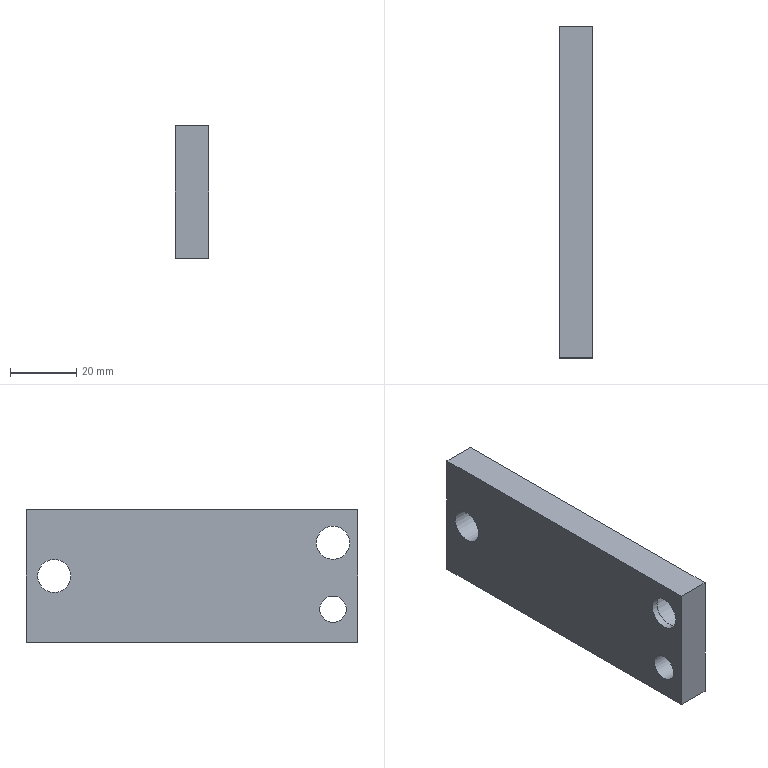Component | NX | DRILL_JIG_PLATE | 1 solid | 13 faces | box 10 x 100 x 40 mm | volume 37387 mm3 | plane 7 | cylinder 5 | cone 1 | commonest cylinder face diameters 10 x2 13 x1 8 x1 4 x1
STEP:
#1=CARTESIAN_POINT('',(0.,0.,0.));
#2=DIRECTION('',(0.,0.,1.));
#3=DIRECTION('',(1.,0.,0.));
#4=AXIS2_PLACEMENT_3D('',#1,#2,#3);
#5=CARTESIAN_POINT('',(49.511,37.872,50.));
#6=VERTEX_POINT('',#5);
#7=CARTESIAN_POINT('',(49.511,37.872,10.));
#8=VERTEX_POINT('',#7);
#9=CARTESIAN_POINT('',(49.511,37.872,50.));
#10=DIRECTION('',(0.,-0.,-1.));
#11=VECTOR('',#10,1.);
#12=LINE('',#9,#11);
#13=CARTESIAN_POINT('',(59.511,37.872,50.));
#14=DIRECTION('',(0.,1.,-0.));
#15=DIRECTION('',(0.,0.,1.));
#16=AXIS2_PLACEMENT_3D('',#13,#14,#15);
#17=PLANE('',#16);
#18=CARTESIAN_POINT('',(0.,-10.));
#19=DIRECTION('',(-1.,0.));
#20=VECTOR('',#19,1.);
#21=LINE('',#18,#20);
#22=(GEOMETRIC_REPRESENTATION_CONTEXT(2)PARAMETRIC_REPRESENTATION_CONTEXT()REPRESENTATION_CONTEXT('',''));
#23=DEFINITIONAL_REPRESENTATION('',(#21),#22);
#24=PCURVE('',#17,#23);
#25=CARTESIAN_POINT('',(49.511,37.872,10.));
#26=DIRECTION('',(1.,0.,0.));
#27=DIRECTION('',(0.,1.,0.));
#28=AXIS2_PLACEMENT_3D('',#25,#26,#27);
#29=PLANE('',#28);
#30=CARTESIAN_POINT('',(0.,40.));
#31=DIRECTION('',(-0.,-1.));
#32=VECTOR('',#31,1.);
#33=LINE('',#30,#32);
#34=(GEOMETRIC_REPRESENTATION_CONTEXT(2)PARAMETRIC_REPRESENTATION_CONTEXT()REPRESENTATION_CONTEXT('',''));
#35=DEFINITIONAL_REPRESENTATION('',(#33),#34);
#36=PCURVE('',#29,#35);
#37=SURFACE_CURVE('',#12,(#24,#36),.PCURVE_S1.);
#38=EDGE_CURVE('',#6,#8,#37,.T.);
#39=ORIENTED_EDGE('',*,*,#38,.T.);
#40=CARTESIAN_POINT('',(59.511,37.872,10.));
#41=VERTEX_POINT('',#40);
#42=CARTESIAN_POINT('',(59.511,37.872,10.));
#43=DIRECTION('',(-1.,0.,0.));
#44=VECTOR('',#43,1.);
#45=LINE('',#42,#44);
#46=CARTESIAN_POINT('',(-40.,0.));
#47=DIRECTION('',(0.,-1.));
#48=VECTOR('',#47,1.);
#49=LINE('',#46,#48);
#50=(GEOMETRIC_REPRESENTATION_CONTEXT(2)PARAMETRIC_REPRESENTATION_CONTEXT()REPRESENTATION_CONTEXT('',''));
#51=DEFINITIONAL_REPRESENTATION('',(#49),#50);
#52=PCURVE('',#17,#51);
#53=CARTESIAN_POINT('',(59.511,37.872,10.));
#54=DIRECTION('',(0.,0.,1.));
#55=DIRECTION('',(1.,0.,0.));
#56=AXIS2_PLACEMENT_3D('',#53,#54,#55);
#57=PLANE('',#56);
#58=CARTESIAN_POINT('',(0.,0.));
#59=DIRECTION('',(-1.,0.));
#60=VECTOR('',#59,1.);
#61=LINE('',#58,#60);
#62=(GEOMETRIC_REPRESENTATION_CONTEXT(2)PARAMETRIC_REPRESENTATION_CONTEXT()REPRESENTATION_CONTEXT('',''));
#63=DEFINITIONAL_REPRESENTATION('',(#61),#62);
#64=PCURVE('',#57,#63);
#65=SURFACE_CURVE('',#45,(#52,#64),.PCURVE_S1.);
#66=EDGE_CURVE('',#41,#8,#65,.T.);
#67=ORIENTED_EDGE('',*,*,#66,.F.);
#68=CARTESIAN_POINT('',(59.511,37.872,50.));
#69=VERTEX_POINT('',#68);
#70=CARTESIAN_POINT('',(59.511,37.872,50.));
#71=DIRECTION('',(0.,-0.,-1.));
#72=VECTOR('',#71,1.);
#73=LINE('',#70,#72);
#74=CARTESIAN_POINT('',(0.,0.));
#75=DIRECTION('',(-1.,0.));
#76=VECTOR('',#75,1.);
#77=LINE('',#74,#76);
#78=(GEOMETRIC_REPRESENTATION_CONTEXT(2)PARAMETRIC_REPRESENTATION_CONTEXT()REPRESENTATION_CONTEXT('',''));
#79=DEFINITIONAL_REPRESENTATION('',(#77),#78);
#80=PCURVE('',#17,#79);
#81=CARTESIAN_POINT('',(59.511,37.872,10.));
#82=DIRECTION('',(1.,0.,0.));
#83=DIRECTION('',(0.,1.,0.));
#84=AXIS2_PLACEMENT_3D('',#81,#82,#83);
#85=PLANE('',#84);
#86=CARTESIAN_POINT('',(0.,40.));
#87=DIRECTION('',(-0.,-1.));
#88=VECTOR('',#87,1.);
#89=LINE('',#86,#88);
#90=(GEOMETRIC_REPRESENTATION_CONTEXT(2)PARAMETRIC_REPRESENTATION_CONTEXT()REPRESENTATION_CONTEXT('',''));
#91=DEFINITIONAL_REPRESENTATION('',(#89),#90);
#92=PCURVE('',#85,#91);
#93=SURFACE_CURVE('',#73,(#80,#92),.PCURVE_S1.);
#94=EDGE_CURVE('',#69,#41,#93,.T.);
#95=ORIENTED_EDGE('',*,*,#94,.F.);
#96=CARTESIAN_POINT('',(59.511,37.872,50.));
#97=DIRECTION('',(-1.,0.,0.));
#98=VECTOR('',#97,1.);
#99=LINE('',#96,#98);
#100=CARTESIAN_POINT('',(0.,0.));
#101=DIRECTION('',(0.,-1.));
#102=VECTOR('',#101,1.);
#103=LINE('',#100,#102);
#104=(GEOMETRIC_REPRESENTATION_CONTEXT(2)PARAMETRIC_REPRESENTATION_CONTEXT()REPRESENTATION_CONTEXT('',''));
#105=DEFINITIONAL_REPRESENTATION('',(#103),#104);
#106=PCURVE('',#17,#105);
#107=CARTESIAN_POINT('',(59.511,137.872,50.));
#108=DIRECTION('',(0.,0.,-1.));
#109=DIRECTION('',(0.,1.,0.));
#110=AXIS2_PLACEMENT_3D('',#107,#108,#109);
#111=PLANE('',#110);
#112=CARTESIAN_POINT('',(-100.,0.));
#113=DIRECTION('',(0.,-1.));
#114=VECTOR('',#113,1.);
#115=LINE('',#112,#114);
#116=(GEOMETRIC_REPRESENTATION_CONTEXT(2)PARAMETRIC_REPRESENTATION_CONTEXT()REPRESENTATION_CONTEXT('',''));
#117=DEFINITIONAL_REPRESENTATION('',(#115),#116);
#118=PCURVE('',#111,#117);
#119=SURFACE_CURVE('',#99,(#106,#118),.PCURVE_S1.);
#120=EDGE_CURVE('',#69,#6,#119,.T.);
#121=ORIENTED_EDGE('',*,*,#120,.T.);
#122=EDGE_LOOP('',(#39,#67,#95,#121));
#123=FACE_BOUND('',#122,.T.);
#124=ADVANCED_FACE('',(#123),#17,.F.);
#125=CARTESIAN_POINT('',(49.511,137.872,10.));
#126=VERTEX_POINT('',#125);
#127=CARTESIAN_POINT('',(49.511,37.872,10.));
#128=DIRECTION('',(0.,1.,0.));
#129=VECTOR('',#128,1.);
#130=LINE('',#127,#129);
#131=CARTESIAN_POINT('',(-10.,0.));
#132=DIRECTION('',(0.,1.));
#133=VECTOR('',#132,1.);
#134=LINE('',#131,#133);
#135=(GEOMETRIC_REPRESENTATION_CONTEXT(2)PARAMETRIC_REPRESENTATION_CONTEXT()REPRESENTATION_CONTEXT('',''));
#136=DEFINITIONAL_REPRESENTATION('',(#134),#135);
#137=PCURVE('',#57,#136);
#138=CARTESIAN_POINT('',(0.,0.));
#139=DIRECTION('',(1.,0.));
#140=VECTOR('',#139,1.);
#141=LINE('',#138,#140);
#142=(GEOMETRIC_REPRESENTATION_CONTEXT(2)PARAMETRIC_REPRESENTATION_CONTEXT()REPRESENTATION_CONTEXT('',''));
#143=DEFINITIONAL_REPRESENTATION('',(#141),#142);
#144=PCURVE('',#29,#143);
#145=SURFACE_CURVE('',#130,(#137,#144),.PCURVE_S1.);
#146=EDGE_CURVE('',#8,#126,#145,.T.);
#147=ORIENTED_EDGE('',*,*,#146,.T.);
#148=CARTESIAN_POINT('',(59.511,137.872,10.));
#149=VERTEX_POINT('',#148);
#150=CARTESIAN_POINT('',(59.511,137.872,10.));
#151=DIRECTION('',(-1.,0.,0.));
#152=VECTOR('',#151,1.);
#153=LINE('',#150,#152);
#154=CARTESIAN_POINT('',(0.,100.));
#155=DIRECTION('',(-1.,0.));
#156=VECTOR('',#155,1.);
#157=LINE('',#154,#156);
#158=(GEOMETRIC_REPRESENTATION_CONTEXT(2)PARAMETRIC_REPRESENTATION_CONTEXT()REPRESENTATION_CONTEXT('',''));
#159=DEFINITIONAL_REPRESENTATION('',(#157),#158);
#160=PCURVE('',#57,#159);
#161=CARTESIAN_POINT('',(59.511,137.872,10.));
#162=DIRECTION('',(0.,-1.,0.));
#163=DIRECTION('',(1.,0.,0.));
#164=AXIS2_PLACEMENT_3D('',#161,#162,#163);
#165=PLANE('',#164);
#166=CARTESIAN_POINT('',(0.,0.));
#167=DIRECTION('',(-1.,0.));
#168=VECTOR('',#167,1.);
#169=LINE('',#166,#168);
#170=(GEOMETRIC_REPRESENTATION_CONTEXT(2)PARAMETRIC_REPRESENTATION_CONTEXT()REPRESENTATION_CONTEXT('',''));
#171=DEFINITIONAL_REPRESENTATION('',(#169),#170);
#172=PCURVE('',#165,#171);
#173=SURFACE_CURVE('',#153,(#160,#172),.PCURVE_S1.);
#174=EDGE_CURVE('',#149,#126,#173,.T.);
#175=ORIENTED_EDGE('',*,*,#174,.F.);
#176=CARTESIAN_POINT('',(59.511,37.872,10.));
#177=DIRECTION('',(0.,1.,0.));
#178=VECTOR('',#177,1.);
#179=LINE('',#176,#178);
#180=CARTESIAN_POINT('',(0.,0.));
#181=DIRECTION('',(0.,1.));
#182=VECTOR('',#181,1.);
#183=LINE('',#180,#182);
#184=(GEOMETRIC_REPRESENTATION_CONTEXT(2)PARAMETRIC_REPRESENTATION_CONTEXT()REPRESENTATION_CONTEXT('',''));
#185=DEFINITIONAL_REPRESENTATION('',(#183),#184);
#186=PCURVE('',#57,#185);
#187=CARTESIAN_POINT('',(0.,0.));
#188=DIRECTION('',(1.,0.));
#189=VECTOR('',#188,1.);
#190=LINE('',#187,#189);
#191=(GEOMETRIC_REPRESENTATION_CONTEXT(2)PARAMETRIC_REPRESENTATION_CONTEXT()REPRESENTATION_CONTEXT('',''));
#192=DEFINITIONAL_REPRESENTATION('',(#190),#191);
#193=PCURVE('',#85,#192);
#194=SURFACE_CURVE('',#179,(#186,#193),.PCURVE_S1.);
#195=EDGE_CURVE('',#41,#149,#194,.T.);
#196=ORIENTED_EDGE('',*,*,#195,.F.);
#197=ORIENTED_EDGE('',*,*,#66,.T.);
#198=EDGE_LOOP('',(#147,#175,#196,#197));
#199=FACE_BOUND('',#198,.T.);
#200=ADVANCED_FACE('',(#199),#57,.F.);
#201=CARTESIAN_POINT('',(49.511,137.872,50.));
#202=VERTEX_POINT('',#201);
#203=CARTESIAN_POINT('',(49.511,137.872,10.));
#204=DIRECTION('',(0.,0.,1.));
#205=VECTOR('',#204,1.);
#206=LINE('',#203,#205);
#207=CARTESIAN_POINT('',(-10.,0.));
#208=DIRECTION('',(0.,1.));
#209=VECTOR('',#208,1.);
#210=LINE('',#207,#209);
#211=(GEOMETRIC_REPRESENTATION_CONTEXT(2)PARAMETRIC_REPRESENTATION_CONTEXT()REPRESENTATION_CONTEXT('',''));
#212=DEFINITIONAL_REPRESENTATION('',(#210),#211);
#213=PCURVE('',#165,#212);
#214=CARTESIAN_POINT('',(100.,0.));
#215=DIRECTION('',(0.,1.));
#216=VECTOR('',#215,1.);
#217=LINE('',#214,#216);
#218=(GEOMETRIC_REPRESENTATION_CONTEXT(2)PARAMETRIC_REPRESENTATION_CONTEXT()REPRESENTATION_CONTEXT('',''));
#219=DEFINITIONAL_REPRESENTATION('',(#217),#218);
#220=PCURVE('',#29,#219);
#221=SURFACE_CURVE('',#206,(#213,#220),.PCURVE_S1.);
#222=EDGE_CURVE('',#126,#202,#221,.T.);
#223=ORIENTED_EDGE('',*,*,#222,.T.);
#224=CARTESIAN_POINT('',(59.511,137.872,50.));
#225=VERTEX_POINT('',#224);
#226=CARTESIAN_POINT('',(59.511,137.872,50.));
#227=DIRECTION('',(-1.,0.,0.));
#228=VECTOR('',#227,1.);
#229=LINE('',#226,#228);
#230=CARTESIAN_POINT('',(0.,40.));
#231=DIRECTION('',(-1.,0.));
#232=VECTOR('',#231,1.);
#233=LINE('',#230,#232);
#234=(GEOMETRIC_REPRESENTATION_CONTEXT(2)PARAMETRIC_REPRESENTATION_CONTEXT()REPRESENTATION_CONTEXT('',''));
#235=DEFINITIONAL_REPRESENTATION('',(#233),#234);
#236=PCURVE('',#165,#235);
#237=CARTESIAN_POINT('',(0.,0.));
#238=DIRECTION('',(0.,-1.));
#239=VECTOR('',#238,1.);
#240=LINE('',#237,#239);
#241=(GEOMETRIC_REPRESENTATION_CONTEXT(2)PARAMETRIC_REPRESENTATION_CONTEXT()REPRESENTATION_CONTEXT('',''));
#242=DEFINITIONAL_REPRESENTATION('',(#240),#241);
#243=PCURVE('',#111,#242);
#244=SURFACE_CURVE('',#229,(#236,#243),.PCURVE_S1.);
#245=EDGE_CURVE('',#225,#202,#244,.T.);
#246=ORIENTED_EDGE('',*,*,#245,.F.);
#247=CARTESIAN_POINT('',(59.511,137.872,10.));
#248=DIRECTION('',(0.,0.,1.));
#249=VECTOR('',#248,1.);
#250=LINE('',#247,#249);
#251=CARTESIAN_POINT('',(0.,0.));
#252=DIRECTION('',(0.,1.));
#253=VECTOR('',#252,1.);
#254=LINE('',#251,#253);
#255=(GEOMETRIC_REPRESENTATION_CONTEXT(2)PARAMETRIC_REPRESENTATION_CONTEXT()REPRESENTATION_CONTEXT('',''));
#256=DEFINITIONAL_REPRESENTATION('',(#254),#255);
#257=PCURVE('',#165,#256);
#258=CARTESIAN_POINT('',(100.,0.));
#259=DIRECTION('',(0.,1.));
#260=VECTOR('',#259,1.);
#261=LINE('',#258,#260);
#262=(GEOMETRIC_REPRESENTATION_CONTEXT(2)PARAMETRIC_REPRESENTATION_CONTEXT()REPRESENTATION_CONTEXT('',''));
#263=DEFINITIONAL_REPRESENTATION('',(#261),#262);
#264=PCURVE('',#85,#263);
#265=SURFACE_CURVE('',#250,(#257,#264),.PCURVE_S1.);
#266=EDGE_CURVE('',#149,#225,#265,.T.);
#267=ORIENTED_EDGE('',*,*,#266,.F.);
#268=ORIENTED_EDGE('',*,*,#174,.T.);
#269=EDGE_LOOP('',(#223,#246,#267,#268));
#270=FACE_BOUND('',#269,.T.);
#271=ADVANCED_FACE('',(#270),#165,.F.);
#272=CARTESIAN_POINT('',(49.511,137.872,50.));
#273=DIRECTION('',(0.,-1.,-0.));
#274=VECTOR('',#273,1.);
#275=LINE('',#272,#274);
#276=CARTESIAN_POINT('',(0.,-10.));
#277=DIRECTION('',(-1.,0.));
#278=VECTOR('',#277,1.);
#279=LINE('',#276,#278);
#280=(GEOMETRIC_REPRESENTATION_CONTEXT(2)PARAMETRIC_REPRESENTATION_CONTEXT()REPRESENTATION_CONTEXT('',''));
#281=DEFINITIONAL_REPRESENTATION('',(#279),#280);
#282=PCURVE('',#111,#281);
#283=CARTESIAN_POINT('',(100.,40.));
#284=DIRECTION('',(-1.,-0.));
#285=VECTOR('',#284,1.);
#286=LINE('',#283,#285);
#287=(GEOMETRIC_REPRESENTATION_CONTEXT(2)PARAMETRIC_REPRESENTATION_CONTEXT()REPRESENTATION_CONTEXT('',''));
#288=DEFINITIONAL_REPRESENTATION('',(#286),#287);
#289=PCURVE('',#29,#288);
#290=SURFACE_CURVE('',#275,(#282,#289),.PCURVE_S1.);
#291=EDGE_CURVE('',#202,#6,#290,.T.);
#292=ORIENTED_EDGE('',*,*,#291,.T.);
#293=ORIENTED_EDGE('',*,*,#120,.F.);
#294=CARTESIAN_POINT('',(59.511,137.872,50.));
#295=DIRECTION('',(0.,-1.,-0.));
#296=VECTOR('',#295,1.);
#297=LINE('',#294,#296);
#298=CARTESIAN_POINT('',(0.,0.));
#299=DIRECTION('',(-1.,0.));
#300=VECTOR('',#299,1.);
#301=LINE('',#298,#300);
#302=(GEOMETRIC_REPRESENTATION_CONTEXT(2)PARAMETRIC_REPRESENTATION_CONTEXT()REPRESENTATION_CONTEXT('',''));
#303=DEFINITIONAL_REPRESENTATION('',(#301),#302);
#304=PCURVE('',#111,#303);
#305=CARTESIAN_POINT('',(100.,40.));
#306=DIRECTION('',(-1.,-0.));
#307=VECTOR('',#306,1.);
#308=LINE('',#305,#307);
#309=(GEOMETRIC_REPRESENTATION_CONTEXT(2)PARAMETRIC_REPRESENTATION_CONTEXT()REPRESENTATION_CONTEXT('',''));
#310=DEFINITIONAL_REPRESENTATION('',(#308),#309);
#311=PCURVE('',#85,#310);
#312=SURFACE_CURVE('',#297,(#304,#311),.PCURVE_S1.);
#313=EDGE_CURVE('',#225,#69,#312,.T.);
#314=ORIENTED_EDGE('',*,*,#313,.F.);
#315=ORIENTED_EDGE('',*,*,#245,.T.);
#316=EDGE_LOOP('',(#292,#293,#314,#315));
#317=FACE_BOUND('',#316,.T.);
#318=ADVANCED_FACE('',(#317),#111,.F.);
#319=CARTESIAN_POINT('',(59.511,117.396,30.));
#320=VERTEX_POINT('',#319);
#321=CARTESIAN_POINT('',(59.511,119.396,30.));
#322=DIRECTION('',(-1.,0.,0.));
#323=DIRECTION('',(0.,-1.,0.));
#324=AXIS2_PLACEMENT_3D('',#321,#322,#323);
#325=CIRCLE('',#324,2.);
#326=CARTESIAN_POINT('',(79.524,20.));
#327=CARTESIAN_POINT('',(79.524,23.464));
#328=CARTESIAN_POINT('',(82.524,21.732));
#329=CARTESIAN_POINT('',(85.524,20.));
#330=CARTESIAN_POINT('',(82.524,18.268));
#331=CARTESIAN_POINT('',(79.524,16.536));
#332=CARTESIAN_POINT('',(79.524,20.));
#333=(BOUNDED_CURVE()B_SPLINE_CURVE(2,(#326,#327,#328,#329,#330,#331,#332),.UNSPECIFIED.,.T.,.F.)B_SPLINE_CURVE_WITH_KNOTS((1,2,2,2,2,1),(-2.094,0.,2.094,4.189,6.283,8.378),.UNSPECIFIED.)CURVE()GEOMETRIC_REPRESENTATION_ITEM()RATIONAL_B_SPLINE_CURVE((1.,0.5,1.,0.5,1.,0.5,1.))REPRESENTATION_ITEM(''));
#334=(GEOMETRIC_REPRESENTATION_CONTEXT(2)PARAMETRIC_REPRESENTATION_CONTEXT()REPRESENTATION_CONTEXT('',''));
#335=DEFINITIONAL_REPRESENTATION('',(#333),#334);
#336=PCURVE('',#85,#335);
#337=CARTESIAN_POINT('',(59.511,119.396,30.));
#338=DIRECTION('',(-1.,0.,0.));
#339=DIRECTION('',(0.,-1.,0.));
#340=AXIS2_PLACEMENT_3D('',#337,#338,#339);
#341=CYLINDRICAL_SURFACE('',#340,2.);
#342=CARTESIAN_POINT('',(0.,0.));
#343=DIRECTION('',(1.,0.));
#344=VECTOR('',#343,1.);
#345=LINE('',#342,#344);
#346=(GEOMETRIC_REPRESENTATION_CONTEXT(2)PARAMETRIC_REPRESENTATION_CONTEXT()REPRESENTATION_CONTEXT('',''));
#347=DEFINITIONAL_REPRESENTATION('',(#345),#346);
#348=PCURVE('',#341,#347);
#349=SURFACE_CURVE('',#325,(#336,#348),.PCURVE_S1.);
#350=EDGE_CURVE('',#320,#320,#349,.T.);
#351=ORIENTED_EDGE('',*,*,#350,.T.);
#352=EDGE_LOOP('',(#351));
#353=FACE_BOUND('',#352,.T.);
#354=CARTESIAN_POINT('',(59.511,134.396,30.));
#355=VERTEX_POINT('',#354);
#356=CARTESIAN_POINT('',(59.511,129.396,30.));
#357=DIRECTION('',(1.,0.,0.));
#358=DIRECTION('',(0.,1.,0.));
#359=AXIS2_PLACEMENT_3D('',#356,#357,#358);
#360=CIRCLE('',#359,5.);
#361=CARTESIAN_POINT('',(91.524,20.));
#362=DIRECTION('',(1.,0.));
#363=AXIS2_PLACEMENT_2D('',#361,#362);
#364=CIRCLE('',#363,5.);
#365=(GEOMETRIC_REPRESENTATION_CONTEXT(2)PARAMETRIC_REPRESENTATION_CONTEXT()REPRESENTATION_CONTEXT('',''));
#366=DEFINITIONAL_REPRESENTATION('',(#364),#365);
#367=PCURVE('',#85,#366);
#368=CARTESIAN_POINT('',(14.511,129.396,30.));
#369=DIRECTION('',(1.,0.,0.));
#370=DIRECTION('',(0.,1.,0.));
#371=AXIS2_PLACEMENT_3D('',#368,#369,#370);
#372=CYLINDRICAL_SURFACE('',#371,5.);
#373=CARTESIAN_POINT('',(0.,45.));
#374=DIRECTION('',(1.,0.));
#375=VECTOR('',#374,1.);
#376=LINE('',#373,#375);
#377=(GEOMETRIC_REPRESENTATION_CONTEXT(2)PARAMETRIC_REPRESENTATION_CONTEXT()REPRESENTATION_CONTEXT('',''));
#378=DEFINITIONAL_REPRESENTATION('',(#376),#377);
#379=PCURVE('',#372,#378);
#380=SURFACE_CURVE('',#360,(#367,#379),.PCURVE_S1.);
#381=EDGE_CURVE('',#355,#355,#380,.T.);
#382=ORIENTED_EDGE('',*,*,#381,.F.);
#383=EDGE_LOOP('',(#382));
#384=FACE_BOUND('',#383,.T.);
#385=CARTESIAN_POINT('',(59.511,49.372,20.));
#386=VERTEX_POINT('',#385);
#387=CARTESIAN_POINT('',(59.511,45.372,20.));
#388=DIRECTION('',(1.,0.,0.));
#389=DIRECTION('',(0.,1.,0.));
#390=AXIS2_PLACEMENT_3D('',#387,#388,#389);
#391=CIRCLE('',#390,4.);
#392=CARTESIAN_POINT('',(7.5,10.));
#393=DIRECTION('',(1.,0.));
#394=AXIS2_PLACEMENT_2D('',#392,#393);
#395=CIRCLE('',#394,4.);
#396=(GEOMETRIC_REPRESENTATION_CONTEXT(2)PARAMETRIC_REPRESENTATION_CONTEXT()REPRESENTATION_CONTEXT('',''));
#397=DEFINITIONAL_REPRESENTATION('',(#395),#396);
#398=PCURVE('',#85,#397);
#399=CARTESIAN_POINT('',(14.511,45.372,20.));
#400=DIRECTION('',(1.,0.,0.));
#401=DIRECTION('',(0.,1.,0.));
#402=AXIS2_PLACEMENT_3D('',#399,#400,#401);
#403=CYLINDRICAL_SURFACE('',#402,4.);
#404=CARTESIAN_POINT('',(0.,45.));
#405=DIRECTION('',(1.,0.));
#406=VECTOR('',#405,1.);
#407=LINE('',#404,#406);
#408=(GEOMETRIC_REPRESENTATION_CONTEXT(2)PARAMETRIC_REPRESENTATION_CONTEXT()REPRESENTATION_CONTEXT('',''));
#409=DEFINITIONAL_REPRESENTATION('',(#407),#408);
#410=PCURVE('',#403,#409);
#411=SURFACE_CURVE('',#391,(#398,#410),.PCURVE_S1.);
#412=EDGE_CURVE('',#386,#386,#411,.T.);
#413=ORIENTED_EDGE('',*,*,#412,.F.);
#414=EDGE_LOOP('',(#413));
#415=FACE_BOUND('',#414,.T.);
#416=CARTESIAN_POINT('',(59.511,38.872,40.));
#417=VERTEX_POINT('',#416);
#418=CARTESIAN_POINT('',(59.511,45.372,40.));
#419=DIRECTION('',(-1.,0.,0.));
#420=DIRECTION('',(0.,-1.,0.));
#421=AXIS2_PLACEMENT_3D('',#418,#419,#420);
#422=CIRCLE('',#421,6.5);
#423=CARTESIAN_POINT('',(1.,30.));
#424=CARTESIAN_POINT('',(1.,41.258));
#425=CARTESIAN_POINT('',(10.75,35.629));
#426=CARTESIAN_POINT('',(20.5,30.));
#427=CARTESIAN_POINT('',(10.75,24.371));
#428=CARTESIAN_POINT('',(1.,18.742));
#429=CARTESIAN_POINT('',(1.,30.));
#430=(BOUNDED_CURVE()B_SPLINE_CURVE(2,(#423,#424,#425,#426,#427,#428,#429),.UNSPECIFIED.,.T.,.F.)B_SPLINE_CURVE_WITH_KNOTS((1,2,2,2,2,1),(-2.094,0.,2.094,4.189,6.283,8.378),.UNSPECIFIED.)CURVE()GEOMETRIC_REPRESENTATION_ITEM()RATIONAL_B_SPLINE_CURVE((1.,0.5,1.,0.5,1.,0.5,1.))REPRESENTATION_ITEM(''));
#431=(GEOMETRIC_REPRESENTATION_CONTEXT(2)PARAMETRIC_REPRESENTATION_CONTEXT()REPRESENTATION_CONTEXT('',''));
#432=DEFINITIONAL_REPRESENTATION('',(#430),#431);
#433=PCURVE('',#85,#432);
#434=CARTESIAN_POINT('',(59.511,45.372,40.));
#435=DIRECTION('',(-1.,0.,0.));
#436=DIRECTION('',(0.,-1.,0.));
#437=AXIS2_PLACEMENT_3D('',#434,#435,#436);
#438=CYLINDRICAL_SURFACE('',#437,6.5);
#439=CARTESIAN_POINT('',(0.,0.));
#440=DIRECTION('',(1.,0.));
#441=VECTOR('',#440,1.);
#442=LINE('',#439,#441);
#443=(GEOMETRIC_REPRESENTATION_CONTEXT(2)PARAMETRIC_REPRESENTATION_CONTEXT()REPRESENTATION_CONTEXT('',''));
#444=DEFINITIONAL_REPRESENTATION('',(#442),#443);
#445=PCURVE('',#438,#444);
#446=SURFACE_CURVE('',#422,(#433,#445),.PCURVE_S1.);
#447=EDGE_CURVE('',#417,#417,#446,.T.);
#448=ORIENTED_EDGE('',*,*,#447,.T.);
#449=EDGE_LOOP('',(#448));
#450=FACE_BOUND('',#449,.T.);
#451=ORIENTED_EDGE('',*,*,#94,.T.);
#452=ORIENTED_EDGE('',*,*,#195,.T.);
#453=ORIENTED_EDGE('',*,*,#266,.T.);
#454=ORIENTED_EDGE('',*,*,#313,.T.);
#455=EDGE_LOOP('',(#451,#452,#453,#454));
#456=FACE_BOUND('',#455,.T.);
#457=ADVANCED_FACE('',(#353,#384,#415,#450,#456),#85,.T.);
#458=CARTESIAN_POINT('',(49.511,134.396,30.));
#459=VERTEX_POINT('',#458);
#460=CARTESIAN_POINT('',(49.511,129.396,30.));
#461=DIRECTION('',(1.,0.,0.));
#462=DIRECTION('',(0.,1.,0.));
#463=AXIS2_PLACEMENT_3D('',#460,#461,#462);
#464=CIRCLE('',#463,5.);
#465=CARTESIAN_POINT('',(91.524,20.));
#466=DIRECTION('',(1.,0.));
#467=AXIS2_PLACEMENT_2D('',#465,#466);
#468=CIRCLE('',#467,5.);
#469=(GEOMETRIC_REPRESENTATION_CONTEXT(2)PARAMETRIC_REPRESENTATION_CONTEXT()REPRESENTATION_CONTEXT('',''));
#470=DEFINITIONAL_REPRESENTATION('',(#468),#469);
#471=PCURVE('',#29,#470);
#472=CARTESIAN_POINT('',(0.,35.));
#473=DIRECTION('',(1.,0.));
#474=VECTOR('',#473,1.);
#475=LINE('',#472,#474);
#476=(GEOMETRIC_REPRESENTATION_CONTEXT(2)PARAMETRIC_REPRESENTATION_CONTEXT()REPRESENTATION_CONTEXT('',''));
#477=DEFINITIONAL_REPRESENTATION('',(#475),#476);
#478=PCURVE('',#372,#477);
#479=SURFACE_CURVE('',#464,(#471,#478),.PCURVE_S1.);
#480=EDGE_CURVE('',#459,#459,#479,.T.);
#481=ORIENTED_EDGE('',*,*,#480,.T.);
#482=EDGE_LOOP('',(#481));
#483=FACE_BOUND('',#482,.T.);
#484=CARTESIAN_POINT('',(49.511,49.372,20.));
#485=VERTEX_POINT('',#484);
#486=CARTESIAN_POINT('',(49.511,45.372,20.));
#487=DIRECTION('',(1.,0.,0.));
#488=DIRECTION('',(0.,1.,0.));
#489=AXIS2_PLACEMENT_3D('',#486,#487,#488);
#490=CIRCLE('',#489,4.);
#491=CARTESIAN_POINT('',(7.5,10.));
#492=DIRECTION('',(1.,0.));
#493=AXIS2_PLACEMENT_2D('',#491,#492);
#494=CIRCLE('',#493,4.);
#495=(GEOMETRIC_REPRESENTATION_CONTEXT(2)PARAMETRIC_REPRESENTATION_CONTEXT()REPRESENTATION_CONTEXT('',''));
#496=DEFINITIONAL_REPRESENTATION('',(#494),#495);
#497=PCURVE('',#29,#496);
#498=CARTESIAN_POINT('',(0.,35.));
#499=DIRECTION('',(1.,0.));
#500=VECTOR('',#499,1.);
#501=LINE('',#498,#500);
#502=(GEOMETRIC_REPRESENTATION_CONTEXT(2)PARAMETRIC_REPRESENTATION_CONTEXT()REPRESENTATION_CONTEXT('',''));
#503=DEFINITIONAL_REPRESENTATION('',(#501),#502);
#504=PCURVE('',#403,#503);
#505=SURFACE_CURVE('',#490,(#497,#504),.PCURVE_S1.);
#506=EDGE_CURVE('',#485,#485,#505,.T.);
#507=ORIENTED_EDGE('',*,*,#506,.T.);
#508=EDGE_LOOP('',(#507));
#509=FACE_BOUND('',#508,.T.);
#510=CARTESIAN_POINT('',(49.511,50.372,40.));
#511=VERTEX_POINT('',#510);
#512=CARTESIAN_POINT('',(49.511,40.372,40.));
#513=VERTEX_POINT('',#512);
#514=CARTESIAN_POINT('',(49.511,45.372,40.));
#515=DIRECTION('',(1.,0.,0.));
#516=DIRECTION('',(0.,1.,0.));
#517=AXIS2_PLACEMENT_3D('',#514,#515,#516);
#518=CIRCLE('',#517,5.);
#519=CARTESIAN_POINT('',(7.5,30.));
#520=DIRECTION('',(1.,0.));
#521=AXIS2_PLACEMENT_2D('',#519,#520);
#522=CIRCLE('',#521,5.);
#523=(GEOMETRIC_REPRESENTATION_CONTEXT(2)PARAMETRIC_REPRESENTATION_CONTEXT()REPRESENTATION_CONTEXT('',''));
#524=DEFINITIONAL_REPRESENTATION('',(#522),#523);
#525=PCURVE('',#29,#524);
#526=CARTESIAN_POINT('',(39.511,45.372,40.));
#527=DIRECTION('',(-1.,0.,0.));
#528=DIRECTION('',(0.,-1.,0.));
#529=AXIS2_PLACEMENT_3D('',#526,#527,#528);
#530=CYLINDRICAL_SURFACE('',#529,5.);
#531=CARTESIAN_POINT('',(3.142,-10.));
#532=DIRECTION('',(-1.,0.));
#533=VECTOR('',#532,1.);
#534=LINE('',#531,#533);
#535=(GEOMETRIC_REPRESENTATION_CONTEXT(2)PARAMETRIC_REPRESENTATION_CONTEXT()REPRESENTATION_CONTEXT('',''));
#536=DEFINITIONAL_REPRESENTATION('',(#534),#535);
#537=PCURVE('',#530,#536);
#538=SURFACE_CURVE('',#518,(#525,#537),.PCURVE_S1.);
#539=EDGE_CURVE('',#511,#513,#538,.T.);
#540=ORIENTED_EDGE('',*,*,#539,.T.);
#541=CARTESIAN_POINT('',(49.511,45.372,40.));
#542=DIRECTION('',(1.,0.,0.));
#543=DIRECTION('',(0.,1.,0.));
#544=AXIS2_PLACEMENT_3D('',#541,#542,#543);
#545=CIRCLE('',#544,5.);
#546=CARTESIAN_POINT('',(7.5,30.));
#547=DIRECTION('',(1.,0.));
#548=AXIS2_PLACEMENT_2D('',#546,#547);
#549=CIRCLE('',#548,5.);
#550=(GEOMETRIC_REPRESENTATION_CONTEXT(2)PARAMETRIC_REPRESENTATION_CONTEXT()REPRESENTATION_CONTEXT('',''));
#551=DEFINITIONAL_REPRESENTATION('',(#549),#550);
#552=PCURVE('',#29,#551);
#553=CARTESIAN_POINT('',(9.425,-10.));
#554=DIRECTION('',(-1.,0.));
#555=VECTOR('',#554,1.);
#556=LINE('',#553,#555);
#557=(GEOMETRIC_REPRESENTATION_CONTEXT(2)PARAMETRIC_REPRESENTATION_CONTEXT()REPRESENTATION_CONTEXT('',''));
#558=DEFINITIONAL_REPRESENTATION('',(#556),#557);
#559=PCURVE('',#530,#558);
#560=SURFACE_CURVE('',#545,(#552,#559),.PCURVE_S1.);
#561=EDGE_CURVE('',#513,#511,#560,.T.);
#562=ORIENTED_EDGE('',*,*,#561,.T.);
#563=EDGE_LOOP('',(#540,#562));
#564=FACE_BOUND('',#563,.T.);
#565=ORIENTED_EDGE('',*,*,#38,.F.);
#566=ORIENTED_EDGE('',*,*,#291,.F.);
#567=ORIENTED_EDGE('',*,*,#222,.F.);
#568=ORIENTED_EDGE('',*,*,#146,.F.);
#569=EDGE_LOOP('',(#565,#566,#567,#568));
#570=FACE_BOUND('',#569,.T.);
#571=ADVANCED_FACE('',(#483,#509,#564,#570),#29,.F.);
#572=CARTESIAN_POINT('',(51.511,40.372,40.));
#573=VERTEX_POINT('',#572);
#574=CARTESIAN_POINT('',(51.511,45.372,40.));
#575=DIRECTION('',(1.,0.,0.));
#576=DIRECTION('',(0.,-1.,0.));
#577=AXIS2_PLACEMENT_3D('',#574,#575,#576);
#578=CIRCLE('',#577,5.);
#579=CARTESIAN_POINT('',(6.283,-12.));
#580=DIRECTION('',(-1.,0.));
#581=VECTOR('',#580,1.);
#582=LINE('',#579,#581);
#583=(GEOMETRIC_REPRESENTATION_CONTEXT(2)PARAMETRIC_REPRESENTATION_CONTEXT()REPRESENTATION_CONTEXT('',''));
#584=DEFINITIONAL_REPRESENTATION('',(#582),#583);
#585=PCURVE('',#530,#584);
#586=CARTESIAN_POINT('',(51.511,45.372,40.));
#587=DIRECTION('',(-1.,0.,0.));
#588=DIRECTION('',(0.,-1.,0.));
#589=AXIS2_PLACEMENT_3D('',#586,#587,#588);
#590=PLANE('',#589);
#591=CARTESIAN_POINT('',(5.,0.));
#592=CARTESIAN_POINT('',(5.,-8.66));
#593=CARTESIAN_POINT('',(-2.5,-4.33));
#594=CARTESIAN_POINT('',(-10.,-0.));
#595=CARTESIAN_POINT('',(-2.5,4.33));
#596=CARTESIAN_POINT('',(5.,8.66));
#597=CARTESIAN_POINT('',(5.,0.));
#598=(BOUNDED_CURVE()B_SPLINE_CURVE(2,(#591,#592,#593,#594,#595,#596,#597),.UNSPECIFIED.,.T.,.F.)B_SPLINE_CURVE_WITH_KNOTS((1,2,2,2,2,1),(-2.094,0.,2.094,4.189,6.283,8.378),.UNSPECIFIED.)CURVE()GEOMETRIC_REPRESENTATION_ITEM()RATIONAL_B_SPLINE_CURVE((1.,0.5,1.,0.5,1.,0.5,1.))REPRESENTATION_ITEM(''));
#599=(GEOMETRIC_REPRESENTATION_CONTEXT(2)PARAMETRIC_REPRESENTATION_CONTEXT()REPRESENTATION_CONTEXT('',''));
#600=DEFINITIONAL_REPRESENTATION('',(#598),#599);
#601=PCURVE('',#590,#600);
#602=SURFACE_CURVE('',#578,(#585,#601),.PCURVE_S1.);
#603=EDGE_CURVE('',#573,#573,#602,.T.);
#604=ORIENTED_EDGE('',*,*,#603,.F.);
#605=CARTESIAN_POINT('',(51.511,40.372,40.));
#606=CARTESIAN_POINT('',(49.511,40.372,40.));
#607=B_SPLINE_CURVE_WITH_KNOTS('',1,(#605,#606),.UNSPECIFIED.,.F.,.F.,(2,2),(-12.,-10.),.PIECEWISE_BEZIER_KNOTS.);
#608=CARTESIAN_POINT('',(6.283,0.));
#609=DIRECTION('',(0.,1.));
#610=VECTOR('',#609,1.);
#611=LINE('',#608,#610);
#612=(GEOMETRIC_REPRESENTATION_CONTEXT(2)PARAMETRIC_REPRESENTATION_CONTEXT()REPRESENTATION_CONTEXT('',''));
#613=DEFINITIONAL_REPRESENTATION('',(#611),#612);
#614=PCURVE('',#530,#613);
#615=CARTESIAN_POINT('',(0.,0.));
#616=DIRECTION('',(0.,1.));
#617=VECTOR('',#616,1.);
#618=LINE('',#615,#617);
#619=(GEOMETRIC_REPRESENTATION_CONTEXT(2)PARAMETRIC_REPRESENTATION_CONTEXT()REPRESENTATION_CONTEXT('',''));
#620=DEFINITIONAL_REPRESENTATION('',(#618),#619);
#621=PCURVE('',#530,#620);
#622=SEAM_CURVE('',#607,(#614,#621),.PCURVE_S1.);
#623=EDGE_CURVE('',#573,#513,#622,.T.);
#624=ORIENTED_EDGE('',*,*,#623,.T.);
#625=ORIENTED_EDGE('',*,*,#561,.T.);
#626=ORIENTED_EDGE('',*,*,#539,.T.);
#627=ORIENTED_EDGE('',*,*,#623,.F.);
#628=EDGE_LOOP('',(#604,#624,#625,#626,#627));
#629=FACE_BOUND('',#628,.F.);
#630=ADVANCED_FACE('',(#629),#530,.F.);
#631=ORIENTED_EDGE('',*,*,#603,.F.);
#632=EDGE_LOOP('',(#631));
#633=FACE_BOUND('',#632,.T.);
#634=CARTESIAN_POINT('',(51.511,38.872,40.));
#635=VERTEX_POINT('',#634);
#636=CARTESIAN_POINT('',(51.511,45.372,40.));
#637=DIRECTION('',(1.,0.,0.));
#638=DIRECTION('',(0.,-1.,0.));
#639=AXIS2_PLACEMENT_3D('',#636,#637,#638);
#640=CIRCLE('',#639,6.5);
#641=CARTESIAN_POINT('',(6.5,0.));
#642=CARTESIAN_POINT('',(6.5,-11.258));
#643=CARTESIAN_POINT('',(-3.25,-5.629));
#644=CARTESIAN_POINT('',(-13.,-0.));
#645=CARTESIAN_POINT('',(-3.25,5.629));
#646=CARTESIAN_POINT('',(6.5,11.258));
#647=CARTESIAN_POINT('',(6.5,0.));
#648=(BOUNDED_CURVE()B_SPLINE_CURVE(2,(#641,#642,#643,#644,#645,#646,#647),.UNSPECIFIED.,.T.,.F.)B_SPLINE_CURVE_WITH_KNOTS((1,2,2,2,2,1),(-2.094,0.,2.094,4.189,6.283,8.378),.UNSPECIFIED.)CURVE()GEOMETRIC_REPRESENTATION_ITEM()RATIONAL_B_SPLINE_CURVE((1.,0.5,1.,0.5,1.,0.5,1.))REPRESENTATION_ITEM(''));
#649=(GEOMETRIC_REPRESENTATION_CONTEXT(2)PARAMETRIC_REPRESENTATION_CONTEXT()REPRESENTATION_CONTEXT('',''));
#650=DEFINITIONAL_REPRESENTATION('',(#648),#649);
#651=PCURVE('',#590,#650);
#652=CARTESIAN_POINT('',(6.283,8.));
#653=DIRECTION('',(-1.,0.));
#654=VECTOR('',#653,1.);
#655=LINE('',#652,#654);
#656=(GEOMETRIC_REPRESENTATION_CONTEXT(2)PARAMETRIC_REPRESENTATION_CONTEXT()REPRESENTATION_CONTEXT('',''));
#657=DEFINITIONAL_REPRESENTATION('',(#655),#656);
#658=PCURVE('',#438,#657);
#659=SURFACE_CURVE('',#640,(#651,#658),.PCURVE_S1.);
#660=EDGE_CURVE('',#635,#635,#659,.T.);
#661=ORIENTED_EDGE('',*,*,#660,.T.);
#662=EDGE_LOOP('',(#661));
#663=FACE_BOUND('',#662,.T.);
#664=ADVANCED_FACE('',(#633,#663),#590,.F.);
#665=ORIENTED_EDGE('',*,*,#660,.T.);
#666=CARTESIAN_POINT('',(59.511,38.872,40.));
#667=CARTESIAN_POINT('',(51.511,38.872,40.));
#668=B_SPLINE_CURVE_WITH_KNOTS('',1,(#666,#667),.UNSPECIFIED.,.F.,.F.,(2,2),(0.,8.),.PIECEWISE_BEZIER_KNOTS.);
#669=CARTESIAN_POINT('',(0.,0.));
#670=DIRECTION('',(0.,1.));
#671=VECTOR('',#670,1.);
#672=LINE('',#669,#671);
#673=(GEOMETRIC_REPRESENTATION_CONTEXT(2)PARAMETRIC_REPRESENTATION_CONTEXT()REPRESENTATION_CONTEXT('',''));
#674=DEFINITIONAL_REPRESENTATION('',(#672),#673);
#675=PCURVE('',#438,#674);
#676=CARTESIAN_POINT('',(6.283,0.));
#677=DIRECTION('',(0.,1.));
#678=VECTOR('',#677,1.);
#679=LINE('',#676,#678);
#680=(GEOMETRIC_REPRESENTATION_CONTEXT(2)PARAMETRIC_REPRESENTATION_CONTEXT()REPRESENTATION_CONTEXT('',''));
#681=DEFINITIONAL_REPRESENTATION('',(#679),#680);
#682=PCURVE('',#438,#681);
#683=SEAM_CURVE('',#668,(#675,#682),.PCURVE_S1.);
#684=EDGE_CURVE('',#417,#635,#683,.T.);
#685=ORIENTED_EDGE('',*,*,#684,.F.);
#686=ORIENTED_EDGE('',*,*,#447,.T.);
#687=ORIENTED_EDGE('',*,*,#684,.T.);
#688=EDGE_LOOP('',(#665,#685,#686,#687));
#689=FACE_BOUND('',#688,.F.);
#690=ADVANCED_FACE('',(#689),#438,.F.);
#691=ORIENTED_EDGE('',*,*,#412,.F.);
#692=CARTESIAN_POINT('',(49.511,49.372,20.));
#693=CARTESIAN_POINT('',(59.511,49.372,20.));
#694=B_SPLINE_CURVE_WITH_KNOTS('',1,(#692,#693),.UNSPECIFIED.,.F.,.F.,(2,2),(35.,45.),.PIECEWISE_BEZIER_KNOTS.);
#695=CARTESIAN_POINT('',(0.,0.));
#696=DIRECTION('',(0.,1.));
#697=VECTOR('',#696,1.);
#698=LINE('',#695,#697);
#699=(GEOMETRIC_REPRESENTATION_CONTEXT(2)PARAMETRIC_REPRESENTATION_CONTEXT()REPRESENTATION_CONTEXT('',''));
#700=DEFINITIONAL_REPRESENTATION('',(#698),#699);
#701=PCURVE('',#403,#700);
#702=CARTESIAN_POINT('',(6.283,0.));
#703=DIRECTION('',(0.,1.));
#704=VECTOR('',#703,1.);
#705=LINE('',#702,#704);
#706=(GEOMETRIC_REPRESENTATION_CONTEXT(2)PARAMETRIC_REPRESENTATION_CONTEXT()REPRESENTATION_CONTEXT('',''));
#707=DEFINITIONAL_REPRESENTATION('',(#705),#706);
#708=PCURVE('',#403,#707);
#709=SEAM_CURVE('',#694,(#701,#708),.PCURVE_S1.);
#710=EDGE_CURVE('',#485,#386,#709,.T.);
#711=ORIENTED_EDGE('',*,*,#710,.F.);
#712=ORIENTED_EDGE('',*,*,#506,.T.);
#713=ORIENTED_EDGE('',*,*,#710,.T.);
#714=EDGE_LOOP('',(#691,#711,#712,#713));
#715=FACE_BOUND('',#714,.F.);
#716=ADVANCED_FACE('',(#715),#403,.F.);
#717=ORIENTED_EDGE('',*,*,#381,.F.);
#718=CARTESIAN_POINT('',(49.511,134.396,30.));
#719=CARTESIAN_POINT('',(59.511,134.396,30.));
#720=B_SPLINE_CURVE_WITH_KNOTS('',1,(#718,#719),.UNSPECIFIED.,.F.,.F.,(2,2),(35.,45.),.PIECEWISE_BEZIER_KNOTS.);
#721=CARTESIAN_POINT('',(0.,0.));
#722=DIRECTION('',(0.,1.));
#723=VECTOR('',#722,1.);
#724=LINE('',#721,#723);
#725=(GEOMETRIC_REPRESENTATION_CONTEXT(2)PARAMETRIC_REPRESENTATION_CONTEXT()REPRESENTATION_CONTEXT('',''));
#726=DEFINITIONAL_REPRESENTATION('',(#724),#725);
#727=PCURVE('',#372,#726);
#728=CARTESIAN_POINT('',(6.283,0.));
#729=DIRECTION('',(0.,1.));
#730=VECTOR('',#729,1.);
#731=LINE('',#728,#730);
#732=(GEOMETRIC_REPRESENTATION_CONTEXT(2)PARAMETRIC_REPRESENTATION_CONTEXT()REPRESENTATION_CONTEXT('',''));
#733=DEFINITIONAL_REPRESENTATION('',(#731),#732);
#734=PCURVE('',#372,#733);
#735=SEAM_CURVE('',#720,(#727,#734),.PCURVE_S1.);
#736=EDGE_CURVE('',#459,#355,#735,.T.);
#737=ORIENTED_EDGE('',*,*,#736,.F.);
#738=ORIENTED_EDGE('',*,*,#480,.T.);
#739=ORIENTED_EDGE('',*,*,#736,.T.);
#740=EDGE_LOOP('',(#717,#737,#738,#739));
#741=FACE_BOUND('',#740,.F.);
#742=ADVANCED_FACE('',(#741),#372,.F.);
#743=CARTESIAN_POINT('',(51.511,121.396,30.));
#744=VERTEX_POINT('',#743);
#745=CARTESIAN_POINT('',(51.511,117.396,30.));
#746=VERTEX_POINT('',#745);
#747=CARTESIAN_POINT('',(51.511,119.396,30.));
#748=DIRECTION('',(1.,0.,0.));
#749=DIRECTION('',(0.,-1.,0.));
#750=AXIS2_PLACEMENT_3D('',#747,#748,#749);
#751=CIRCLE('',#750,2.);
#752=CARTESIAN_POINT('',(51.511,119.396,30.));
#753=DIRECTION('',(1.,0.,0.));
#754=DIRECTION('',(0.,1.,0.));
#755=AXIS2_PLACEMENT_3D('',#752,#753,#754);
#756=CONICAL_SURFACE('',#755,2.,1.03);
#757=CARTESIAN_POINT('',(-3.142,0.));
#758=DIRECTION('',(1.,0.));
#759=VECTOR('',#758,1.);
#760=LINE('',#757,#759);
#761=(GEOMETRIC_REPRESENTATION_CONTEXT(2)PARAMETRIC_REPRESENTATION_CONTEXT()REPRESENTATION_CONTEXT('',''));
#762=DEFINITIONAL_REPRESENTATION('',(#760),#761);
#763=PCURVE('',#756,#762);
#764=CARTESIAN_POINT('',(6.283,8.));
#765=DIRECTION('',(-1.,0.));
#766=VECTOR('',#765,1.);
#767=LINE('',#764,#766);
#768=(GEOMETRIC_REPRESENTATION_CONTEXT(2)PARAMETRIC_REPRESENTATION_CONTEXT()REPRESENTATION_CONTEXT('',''));
#769=DEFINITIONAL_REPRESENTATION('',(#767),#768);
#770=PCURVE('',#341,#769);
#771=SURFACE_CURVE('',#751,(#763,#770),.PCURVE_S1.);
#772=EDGE_CURVE('',#744,#746,#771,.T.);
#773=ORIENTED_EDGE('',*,*,#772,.F.);
#774=CARTESIAN_POINT('',(50.309,119.396,30.));
#775=VERTEX_POINT('',#774);
#776=CARTESIAN_POINT('',(50.309,119.396,30.));
#777=CARTESIAN_POINT('',(51.511,121.396,30.));
#778=B_SPLINE_CURVE_WITH_KNOTS('',1,(#776,#777),.UNSPECIFIED.,.F.,.F.,(2,2),(-2.333,0.),.PIECEWISE_BEZIER_KNOTS.);
#779=CARTESIAN_POINT('',(0.,0.));
#780=DIRECTION('',(0.,1.));
#781=VECTOR('',#780,1.);
#782=LINE('',#779,#781);
#783=(GEOMETRIC_REPRESENTATION_CONTEXT(2)PARAMETRIC_REPRESENTATION_CONTEXT()REPRESENTATION_CONTEXT('',''));
#784=DEFINITIONAL_REPRESENTATION('',(#782),#783);
#785=PCURVE('',#756,#784);
#786=CARTESIAN_POINT('',(6.283,0.));
#787=DIRECTION('',(0.,1.));
#788=VECTOR('',#787,1.);
#789=LINE('',#786,#788);
#790=(GEOMETRIC_REPRESENTATION_CONTEXT(2)PARAMETRIC_REPRESENTATION_CONTEXT()REPRESENTATION_CONTEXT('',''));
#791=DEFINITIONAL_REPRESENTATION('',(#789),#790);
#792=PCURVE('',#756,#791);
#793=SEAM_CURVE('',#778,(#785,#792),.PCURVE_S1.);
#794=EDGE_CURVE('',#775,#744,#793,.T.);
#795=ORIENTED_EDGE('',*,*,#794,.F.);
#796=ORIENTED_EDGE('',*,*,#794,.T.);
#797=CARTESIAN_POINT('',(51.511,119.396,30.));
#798=DIRECTION('',(1.,0.,0.));
#799=DIRECTION('',(0.,-1.,0.));
#800=AXIS2_PLACEMENT_3D('',#797,#798,#799);
#801=CIRCLE('',#800,2.);
#802=CARTESIAN_POINT('',(3.142,0.));
#803=DIRECTION('',(1.,0.));
#804=VECTOR('',#803,1.);
#805=LINE('',#802,#804);
#806=(GEOMETRIC_REPRESENTATION_CONTEXT(2)PARAMETRIC_REPRESENTATION_CONTEXT()REPRESENTATION_CONTEXT('',''));
#807=DEFINITIONAL_REPRESENTATION('',(#805),#806);
#808=PCURVE('',#756,#807);
#809=CARTESIAN_POINT('',(6.283,8.));
#810=DIRECTION('',(-1.,0.));
#811=VECTOR('',#810,1.);
#812=LINE('',#809,#811);
#813=(GEOMETRIC_REPRESENTATION_CONTEXT(2)PARAMETRIC_REPRESENTATION_CONTEXT()REPRESENTATION_CONTEXT('',''));
#814=DEFINITIONAL_REPRESENTATION('',(#812),#813);
#815=PCURVE('',#341,#814);
#816=SURFACE_CURVE('',#801,(#808,#815),.PCURVE_S1.);
#817=EDGE_CURVE('',#746,#744,#816,.T.);
#818=ORIENTED_EDGE('',*,*,#817,.F.);
#819=EDGE_LOOP('',(#773,#795,#796,#818));
#820=FACE_BOUND('',#819,.F.);
#821=ADVANCED_FACE('',(#820),#756,.F.);
#822=ORIENTED_EDGE('',*,*,#772,.T.);
#823=CARTESIAN_POINT('',(59.511,117.396,30.));
#824=CARTESIAN_POINT('',(51.511,117.396,30.));
#825=B_SPLINE_CURVE_WITH_KNOTS('',1,(#823,#824),.UNSPECIFIED.,.F.,.F.,(2,2),(0.,8.),.PIECEWISE_BEZIER_KNOTS.);
#826=CARTESIAN_POINT('',(0.,0.));
#827=DIRECTION('',(0.,1.));
#828=VECTOR('',#827,1.);
#829=LINE('',#826,#828);
#830=(GEOMETRIC_REPRESENTATION_CONTEXT(2)PARAMETRIC_REPRESENTATION_CONTEXT()REPRESENTATION_CONTEXT('',''));
#831=DEFINITIONAL_REPRESENTATION('',(#829),#830);
#832=PCURVE('',#341,#831);
#833=CARTESIAN_POINT('',(6.283,0.));
#834=DIRECTION('',(0.,1.));
#835=VECTOR('',#834,1.);
#836=LINE('',#833,#835);
#837=(GEOMETRIC_REPRESENTATION_CONTEXT(2)PARAMETRIC_REPRESENTATION_CONTEXT()REPRESENTATION_CONTEXT('',''));
#838=DEFINITIONAL_REPRESENTATION('',(#836),#837);
#839=PCURVE('',#341,#838);
#840=SEAM_CURVE('',#825,(#832,#839),.PCURVE_S1.);
#841=EDGE_CURVE('',#320,#746,#840,.T.);
#842=ORIENTED_EDGE('',*,*,#841,.F.);
#843=ORIENTED_EDGE('',*,*,#350,.T.);
#844=ORIENTED_EDGE('',*,*,#841,.T.);
#845=ORIENTED_EDGE('',*,*,#817,.T.);
#846=EDGE_LOOP('',(#822,#842,#843,#844,#845));
#847=FACE_BOUND('',#846,.F.);
#848=ADVANCED_FACE('',(#847),#341,.F.);
#849=CLOSED_SHELL('',(#124,#200,#271,#318,#457,#571,#630,#664,#690,#716,#742,#821,#848));
#850=MANIFOLD_SOLID_BREP('',#849);
#851=(LENGTH_UNIT()NAMED_UNIT(*)SI_UNIT(.MILLI.,.METRE.));
#852=UNCERTAINTY_MEASURE_WITH_UNIT(LENGTH_MEASURE(0.000005),#851,'','');
#853=(NAMED_UNIT(*)PLANE_ANGLE_UNIT()SI_UNIT($,.RADIAN.));
#854=(NAMED_UNIT(*)SI_UNIT($,.STERADIAN.)SOLID_ANGLE_UNIT());
#855=(GEOMETRIC_REPRESENTATION_CONTEXT(3)GLOBAL_UNCERTAINTY_ASSIGNED_CONTEXT((#852))GLOBAL_UNIT_ASSIGNED_CONTEXT((#851,#853,#854))REPRESENTATION_CONTEXT('',''));
#856=ADVANCED_BREP_SHAPE_REPRESENTATION('',(#4,#850),#855);